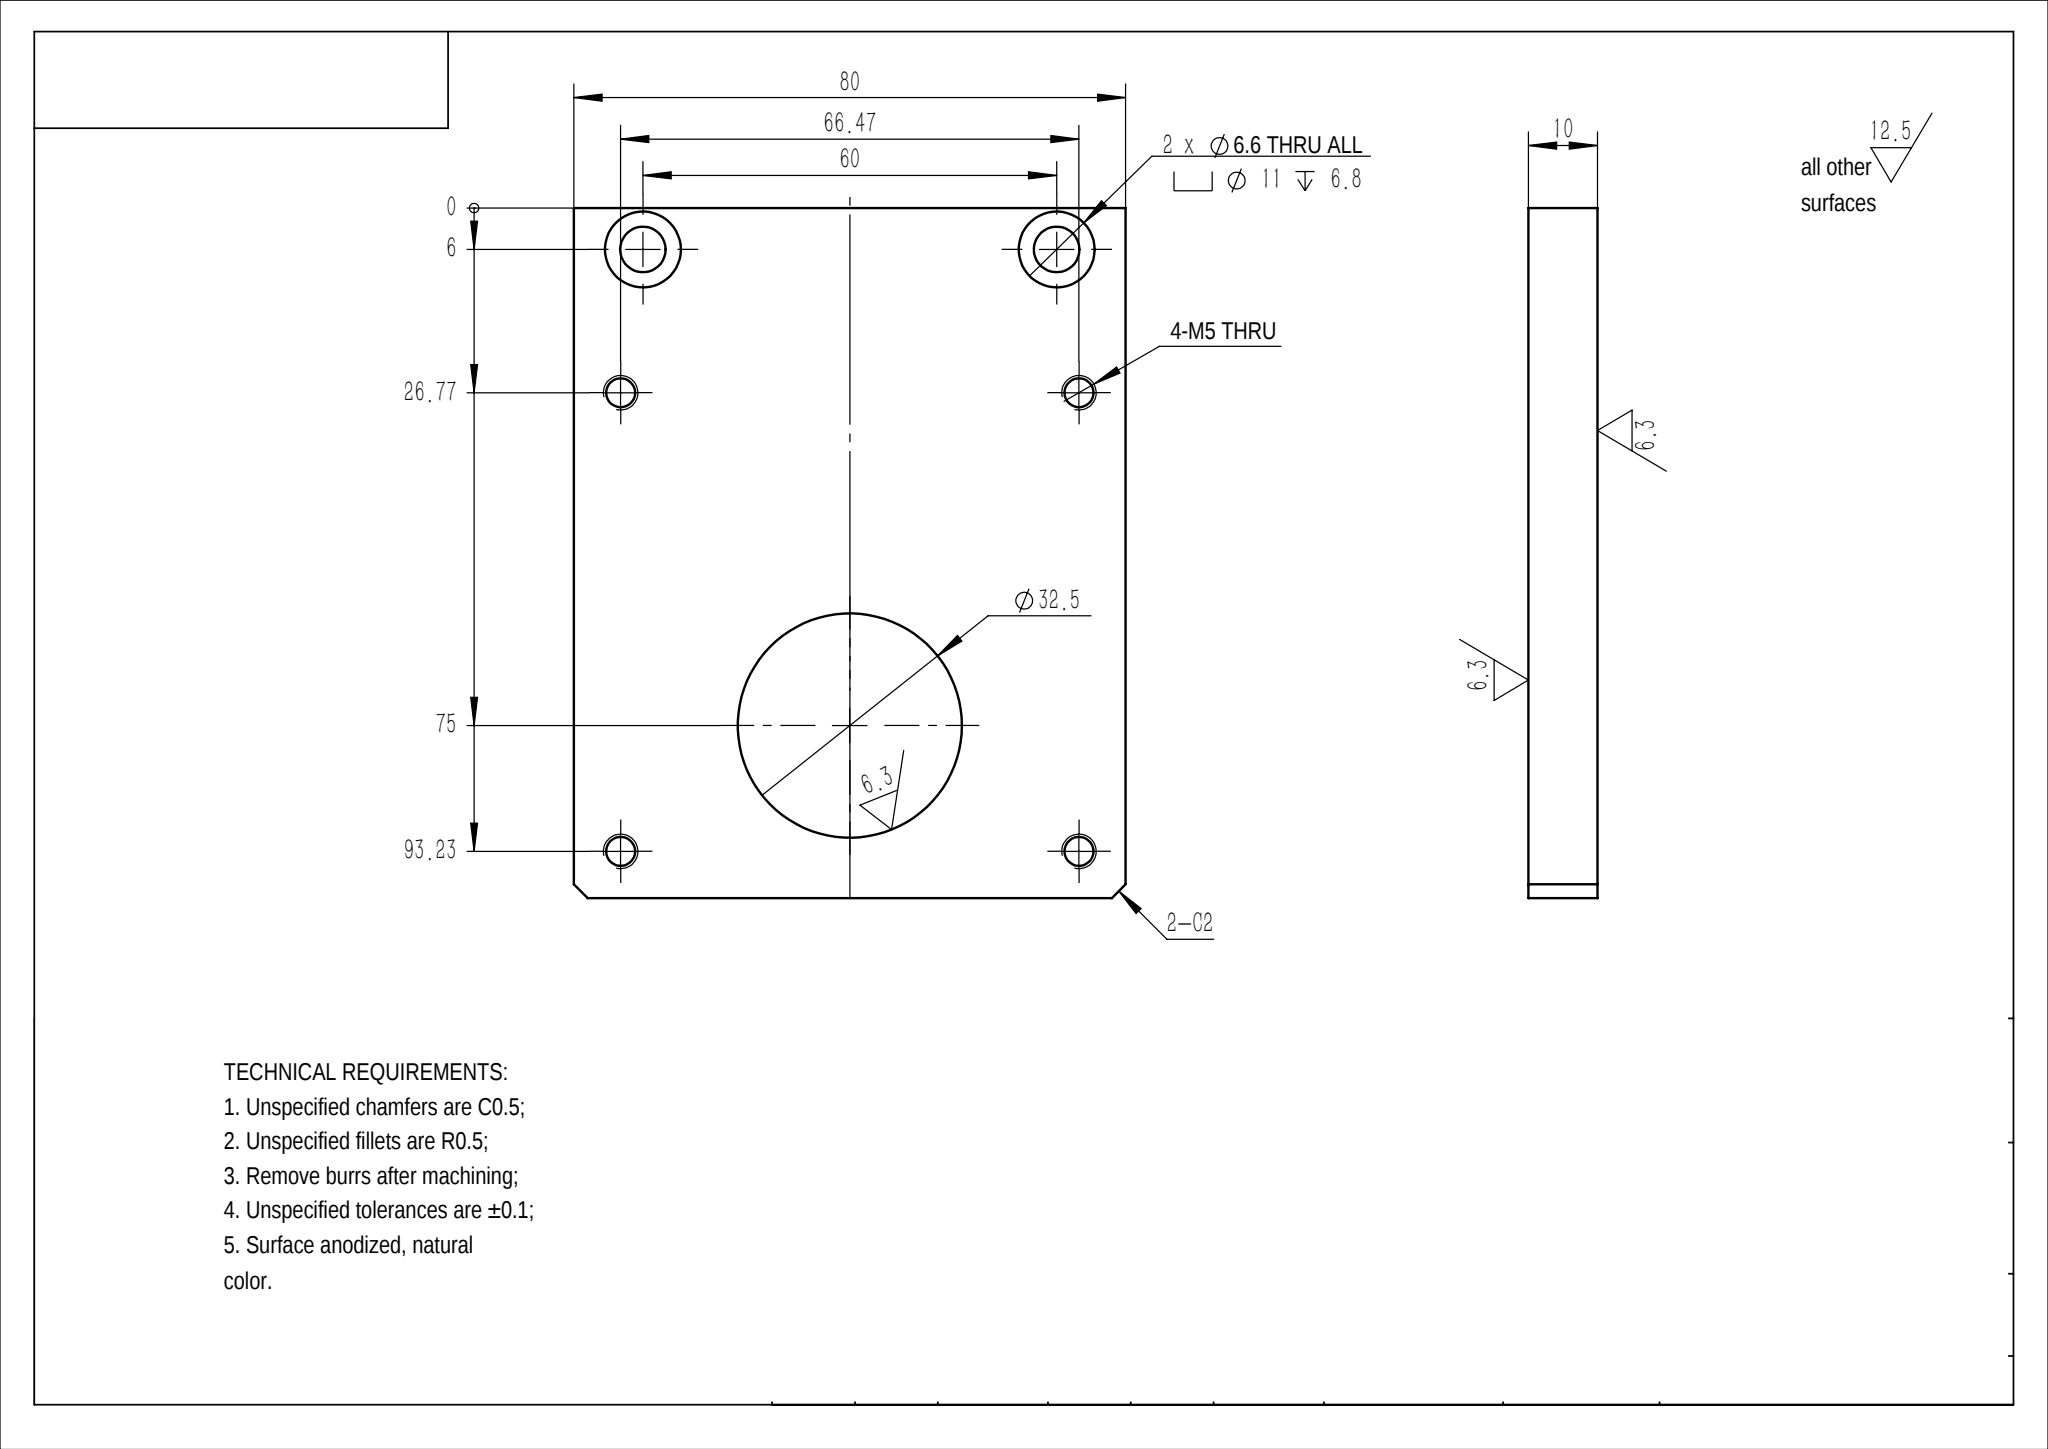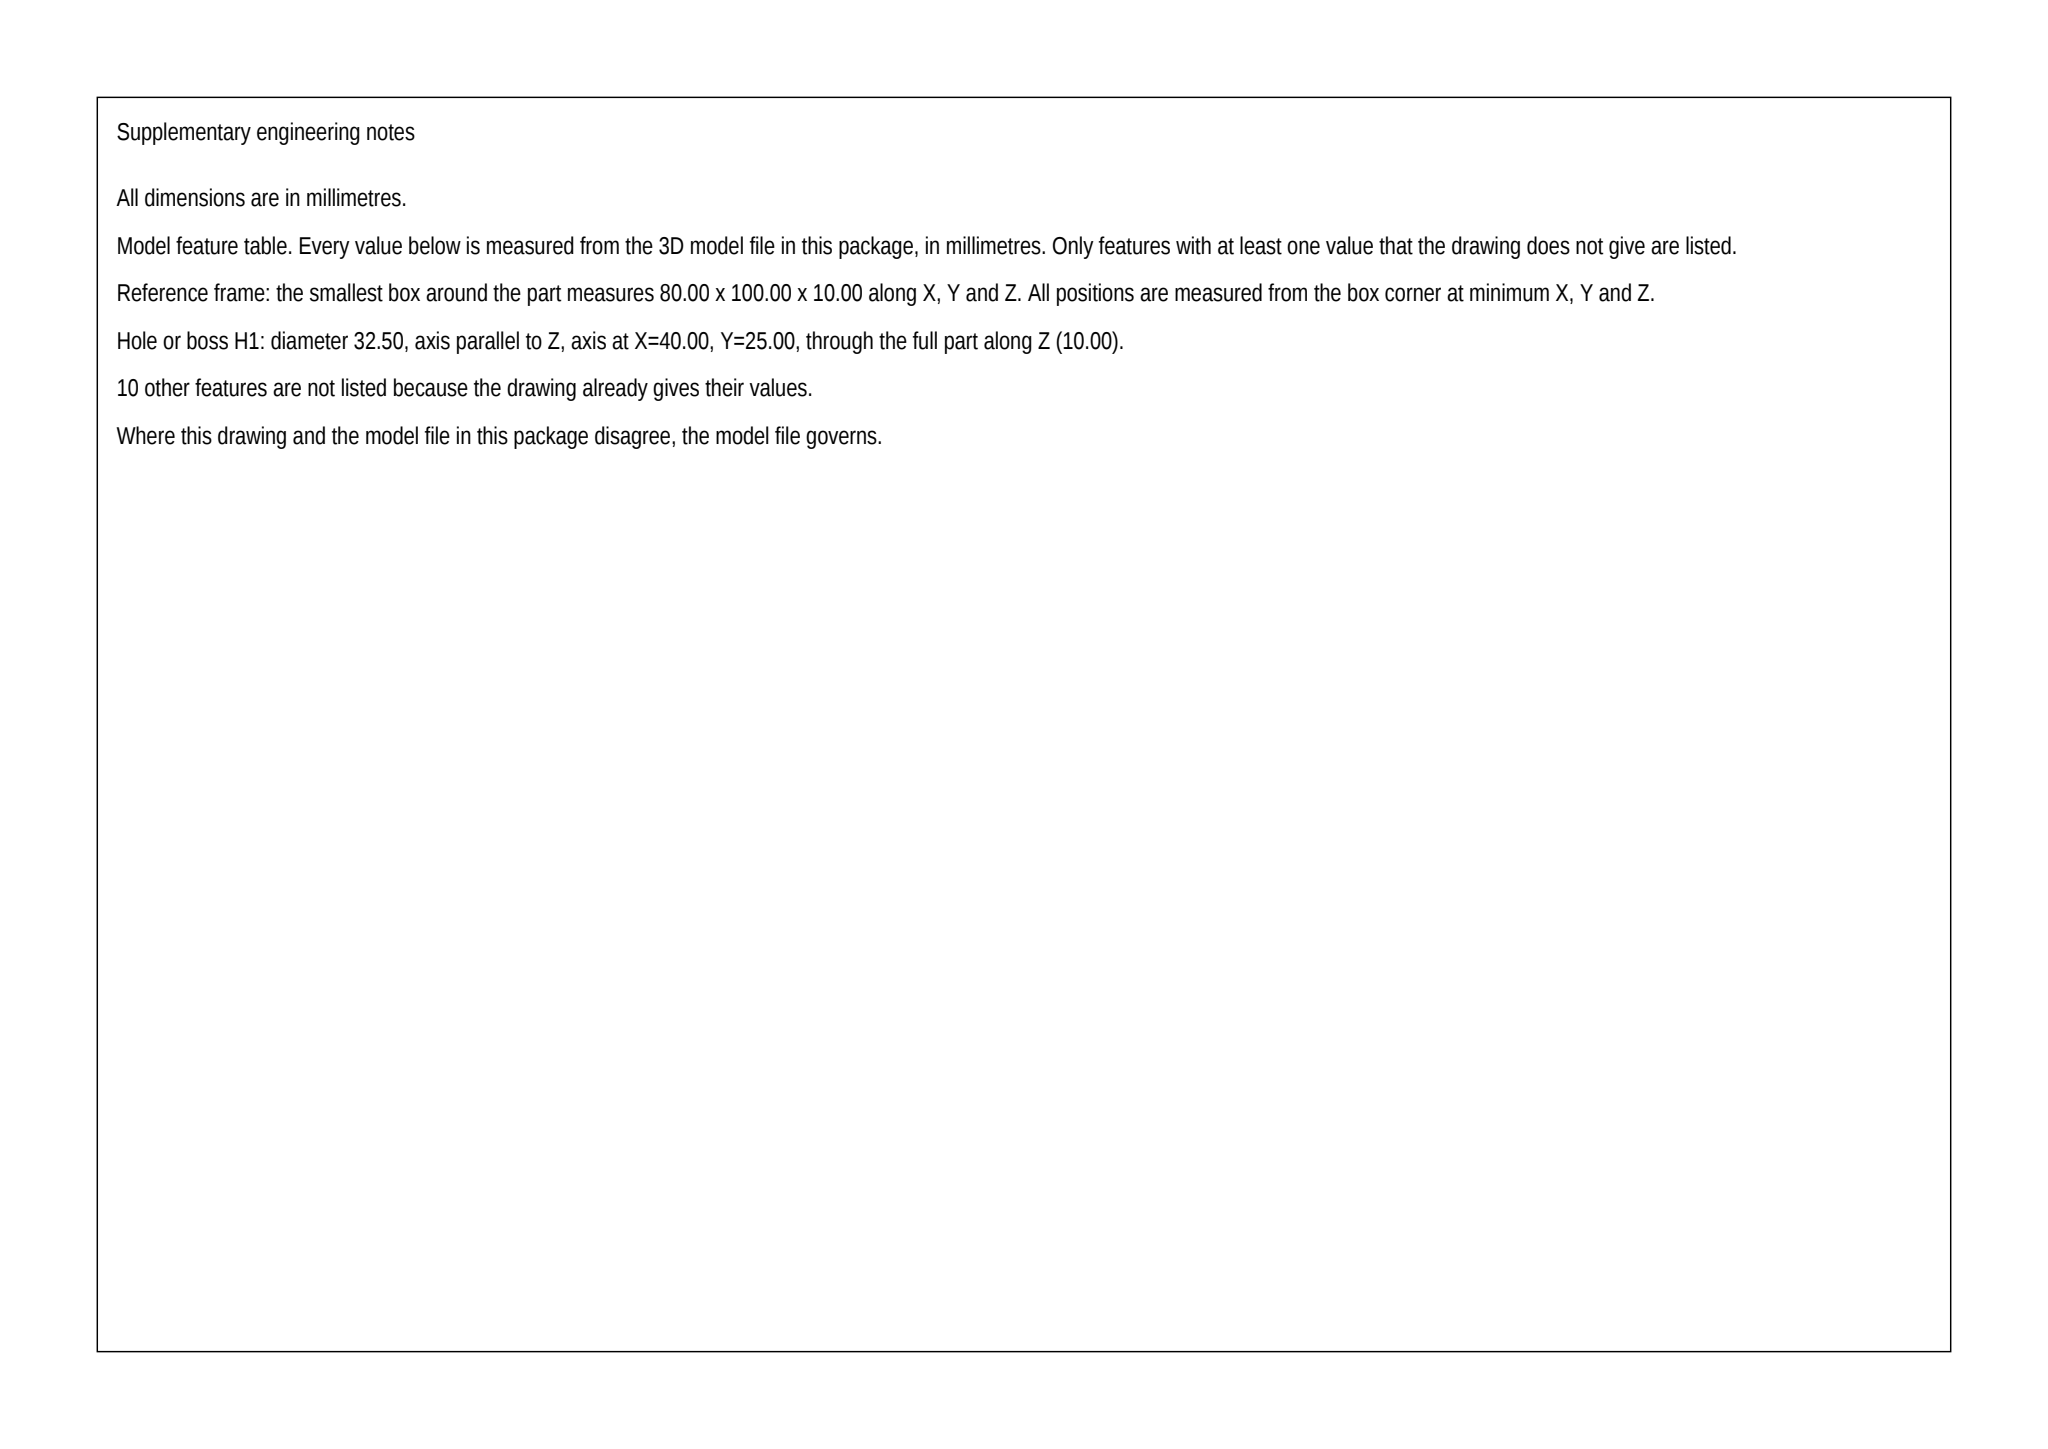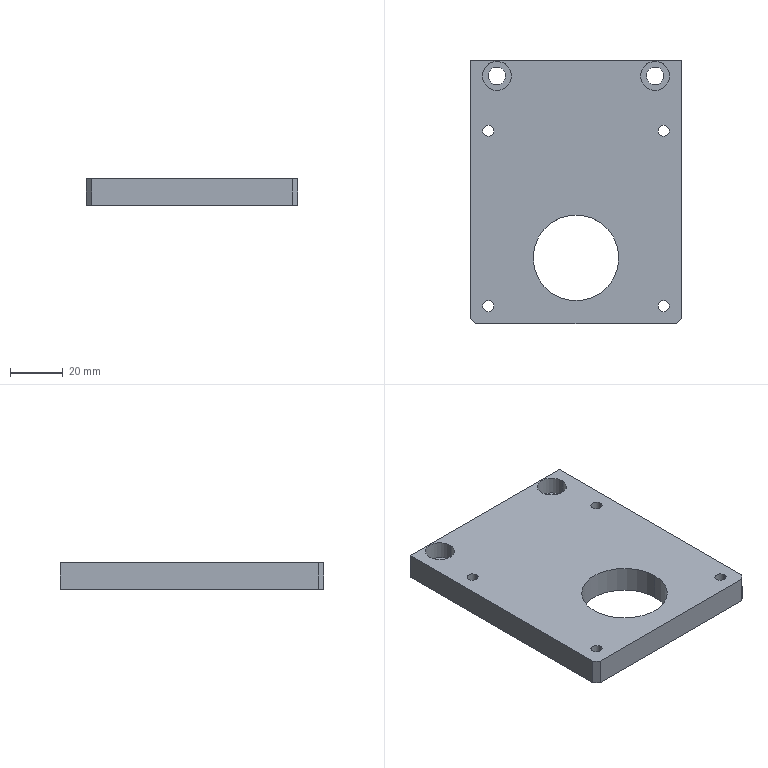Part | SolidWorks | mm | 1 solid | 28 faces | box 80 x 100 x 10 mm | volume 69599 mm3 | cylinder 18 | plane 10 | commonest cylinder face diameters 4.2 x8 11 x4 6.6 x4 32.5 x2
build123d program:
from build123d import *

# Parameters (mm, degrees)
SKETCH1_W                                            = 80
SKETCH1_H                                            = 100
BOSS_EXTRUDE1_DEPTH                                  = 10
SKETCH2_R                                            = 16.25
CUT_EXTRUDE1_DEPTH                                   = 65.807
M5_TAPPED_HOLE1_D                                    = 4.2
CHAMFER1_SIZE                                        = 2
HOLE_SIZE_ACCORDING_TO_TYPE_1_OF_HEXAGON_D           = 6.6
HOLE_SIZE_ACCORDING_TO_TYPE_1_OF_HEXAGON_CBORE_D     = 11
HOLE_SIZE_ACCORDING_TO_TYPE_1_OF_HEXAGON_CBORE_DEPTH = 6.8


with BuildPart() as part:
    # Sketch1 → Boss-Extrude1 (new body)
    with BuildSketch(Plane.XY):
        Rectangle(SKETCH1_W, SKETCH1_H)
    extrude(amount=BOSS_EXTRUDE1_DEPTH)

    # Sketch2 → Cut-Extrude1 (cut, through all)
    with BuildSketch(Plane.XY.offset(10)):
        with Locations((0, -25)):
            Circle(SKETCH2_R)
    extrude(amount=-CUT_EXTRUDE1_DEPTH, mode=Mode.SUBTRACT)

    # M5 Tapped Hole1 (through all)
    with Locations(Plane.XY.offset(10)):
        with Locations((-33.234, 23.234), (-33.234, -43.234), (33.234, -43.234), (33.234, 23.234)):
            Hole(M5_TAPPED_HOLE1_D / 2)

    # Chamfer1
    chamfer1_edges = [part.edges().sort_by_distance(p)[0] for p in [
        (40, -50, 5),
        (-40, -50, 5),
    ]]
    chamfer(chamfer1_edges, length=CHAMFER1_SIZE)

    # Hole Size_According to_Type 1 of Hexagon (through all)
    with Locations(Plane.XY.offset(10)):
        with Locations((-30, 44), (30, 44)):
            CounterBoreHole(HOLE_SIZE_ACCORDING_TO_TYPE_1_OF_HEXAGON_D / 2, HOLE_SIZE_ACCORDING_TO_TYPE_1_OF_HEXAGON_CBORE_D / 2, HOLE_SIZE_ACCORDING_TO_TYPE_1_OF_HEXAGON_CBORE_DEPTH)


solid = part.part
STEP:
#1=CARTESIAN_POINT('',(-35.5,44.,3.2));
#2=VERTEX_POINT('',#1);
#3=CARTESIAN_POINT('',(-24.5,44.,3.2));
#4=VERTEX_POINT('',#3);
#5=CARTESIAN_POINT('',(-30.,44.,3.2));
#6=DIRECTION('',(0.,0.,1.));
#7=DIRECTION('',(1.,0.,0.));
#8=AXIS2_PLACEMENT_3D('',#5,#6,#7);
#9=CIRCLE('',#8,5.5);
#10=EDGE_CURVE('',#2,#4,#9,.T.);
#11=ORIENTED_EDGE('',*,*,#10,.F.);
#12=CARTESIAN_POINT('',(-35.5,44.,10.));
#13=VERTEX_POINT('',#12);
#14=CARTESIAN_POINT('',(-35.5,44.,10.));
#15=DIRECTION('',(0.,0.,1.));
#16=VECTOR('',#15,1000.);
#17=LINE('',#14,#16);
#18=EDGE_CURVE('',#2,#13,#17,.T.);
#19=ORIENTED_EDGE('',*,*,#18,.T.);
#20=CARTESIAN_POINT('',(-24.5,44.,10.));
#21=VERTEX_POINT('',#20);
#22=CARTESIAN_POINT('',(-30.,44.,10.));
#23=DIRECTION('',(0.,0.,1.));
#24=DIRECTION('',(1.,0.,0.));
#25=AXIS2_PLACEMENT_3D('',#22,#23,#24);
#26=CIRCLE('',#25,5.5);
#27=EDGE_CURVE('',#13,#21,#26,.T.);
#28=ORIENTED_EDGE('',*,*,#27,.T.);
#29=CARTESIAN_POINT('',(-24.5,44.,10.));
#30=DIRECTION('',(0.,0.,1.));
#31=VECTOR('',#30,1000.);
#32=LINE('',#29,#31);
#33=EDGE_CURVE('',#4,#21,#32,.T.);
#34=ORIENTED_EDGE('',*,*,#33,.F.);
#35=EDGE_LOOP('',(#11,#19,#28,#34));
#36=FACE_OUTER_BOUND('',#35,.T.);
#37=CARTESIAN_POINT('',(-30.,44.,10.));
#38=DIRECTION('',(0.,0.,1.));
#39=DIRECTION('',(1.,0.,0.));
#40=AXIS2_PLACEMENT_3D('',#37,#38,#39);
#41=CYLINDRICAL_SURFACE('',#40,5.5);
#42=ADVANCED_FACE('',(#36),#41,.F.);
#43=CARTESIAN_POINT('',(-33.3,44.,0.));
#44=VERTEX_POINT('',#43);
#45=CARTESIAN_POINT('',(-26.7,44.,0.));
#46=VERTEX_POINT('',#45);
#47=CARTESIAN_POINT('',(-30.,44.,0.));
#48=DIRECTION('',(0.,0.,1.));
#49=DIRECTION('',(1.,0.,0.));
#50=AXIS2_PLACEMENT_3D('',#47,#48,#49);
#51=CIRCLE('',#50,3.3);
#52=EDGE_CURVE('',#44,#46,#51,.T.);
#53=ORIENTED_EDGE('',*,*,#52,.F.);
#54=CARTESIAN_POINT('',(-33.3,44.,3.2));
#55=VERTEX_POINT('',#54);
#56=CARTESIAN_POINT('',(-33.3,44.,10.));
#57=DIRECTION('',(0.,0.,1.));
#58=VECTOR('',#57,1000.);
#59=LINE('',#56,#58);
#60=EDGE_CURVE('',#44,#55,#59,.T.);
#61=ORIENTED_EDGE('',*,*,#60,.T.);
#62=CARTESIAN_POINT('',(-26.7,44.,3.2));
#63=VERTEX_POINT('',#62);
#64=CARTESIAN_POINT('',(-30.,44.,3.2));
#65=DIRECTION('',(0.,0.,1.));
#66=DIRECTION('',(1.,0.,0.));
#67=AXIS2_PLACEMENT_3D('',#64,#65,#66);
#68=CIRCLE('',#67,3.3);
#69=EDGE_CURVE('',#55,#63,#68,.T.);
#70=ORIENTED_EDGE('',*,*,#69,.T.);
#71=CARTESIAN_POINT('',(-26.7,44.,10.));
#72=DIRECTION('',(0.,0.,1.));
#73=VECTOR('',#72,1000.);
#74=LINE('',#71,#73);
#75=EDGE_CURVE('',#46,#63,#74,.T.);
#76=ORIENTED_EDGE('',*,*,#75,.F.);
#77=EDGE_LOOP('',(#53,#61,#70,#76));
#78=FACE_OUTER_BOUND('',#77,.T.);
#79=CARTESIAN_POINT('',(-30.,44.,10.));
#80=DIRECTION('',(0.,0.,1.));
#81=DIRECTION('',(1.,0.,0.));
#82=AXIS2_PLACEMENT_3D('',#79,#80,#81);
#83=CYLINDRICAL_SURFACE('',#82,3.3);
#84=ADVANCED_FACE('',(#78),#83,.F.);
#85=CARTESIAN_POINT('',(24.5,44.,3.2));
#86=VERTEX_POINT('',#85);
#87=CARTESIAN_POINT('',(35.5,44.,3.2));
#88=VERTEX_POINT('',#87);
#89=CARTESIAN_POINT('',(30.,44.,3.2));
#90=DIRECTION('',(0.,0.,1.));
#91=DIRECTION('',(1.,0.,0.));
#92=AXIS2_PLACEMENT_3D('',#89,#90,#91);
#93=CIRCLE('',#92,5.5);
#94=EDGE_CURVE('',#86,#88,#93,.T.);
#95=ORIENTED_EDGE('',*,*,#94,.F.);
#96=CARTESIAN_POINT('',(24.5,44.,10.));
#97=VERTEX_POINT('',#96);
#98=CARTESIAN_POINT('',(24.5,44.,10.));
#99=DIRECTION('',(0.,0.,1.));
#100=VECTOR('',#99,1000.);
#101=LINE('',#98,#100);
#102=EDGE_CURVE('',#86,#97,#101,.T.);
#103=ORIENTED_EDGE('',*,*,#102,.T.);
#104=CARTESIAN_POINT('',(35.5,44.,10.));
#105=VERTEX_POINT('',#104);
#106=CARTESIAN_POINT('',(30.,44.,10.));
#107=DIRECTION('',(0.,0.,1.));
#108=DIRECTION('',(1.,0.,0.));
#109=AXIS2_PLACEMENT_3D('',#106,#107,#108);
#110=CIRCLE('',#109,5.5);
#111=EDGE_CURVE('',#97,#105,#110,.T.);
#112=ORIENTED_EDGE('',*,*,#111,.T.);
#113=CARTESIAN_POINT('',(35.5,44.,10.));
#114=DIRECTION('',(0.,0.,1.));
#115=VECTOR('',#114,1000.);
#116=LINE('',#113,#115);
#117=EDGE_CURVE('',#88,#105,#116,.T.);
#118=ORIENTED_EDGE('',*,*,#117,.F.);
#119=EDGE_LOOP('',(#95,#103,#112,#118));
#120=FACE_OUTER_BOUND('',#119,.T.);
#121=CARTESIAN_POINT('',(30.,44.,10.));
#122=DIRECTION('',(0.,0.,1.));
#123=DIRECTION('',(1.,0.,0.));
#124=AXIS2_PLACEMENT_3D('',#121,#122,#123);
#125=CYLINDRICAL_SURFACE('',#124,5.5);
#126=ADVANCED_FACE('',(#120),#125,.F.);
#127=CARTESIAN_POINT('',(26.7,44.,0.));
#128=VERTEX_POINT('',#127);
#129=CARTESIAN_POINT('',(33.3,44.,0.));
#130=VERTEX_POINT('',#129);
#131=CARTESIAN_POINT('',(30.,44.,0.));
#132=DIRECTION('',(0.,0.,1.));
#133=DIRECTION('',(1.,0.,0.));
#134=AXIS2_PLACEMENT_3D('',#131,#132,#133);
#135=CIRCLE('',#134,3.3);
#136=EDGE_CURVE('',#128,#130,#135,.T.);
#137=ORIENTED_EDGE('',*,*,#136,.F.);
#138=CARTESIAN_POINT('',(26.7,44.,3.2));
#139=VERTEX_POINT('',#138);
#140=CARTESIAN_POINT('',(26.7,44.,10.));
#141=DIRECTION('',(0.,0.,1.));
#142=VECTOR('',#141,1000.);
#143=LINE('',#140,#142);
#144=EDGE_CURVE('',#128,#139,#143,.T.);
#145=ORIENTED_EDGE('',*,*,#144,.T.);
#146=CARTESIAN_POINT('',(33.3,44.,3.2));
#147=VERTEX_POINT('',#146);
#148=CARTESIAN_POINT('',(30.,44.,3.2));
#149=DIRECTION('',(0.,0.,1.));
#150=DIRECTION('',(1.,0.,0.));
#151=AXIS2_PLACEMENT_3D('',#148,#149,#150);
#152=CIRCLE('',#151,3.3);
#153=EDGE_CURVE('',#139,#147,#152,.T.);
#154=ORIENTED_EDGE('',*,*,#153,.T.);
#155=CARTESIAN_POINT('',(33.3,44.,10.));
#156=DIRECTION('',(0.,0.,1.));
#157=VECTOR('',#156,1000.);
#158=LINE('',#155,#157);
#159=EDGE_CURVE('',#130,#147,#158,.T.);
#160=ORIENTED_EDGE('',*,*,#159,.F.);
#161=EDGE_LOOP('',(#137,#145,#154,#160));
#162=FACE_OUTER_BOUND('',#161,.T.);
#163=CARTESIAN_POINT('',(30.,44.,10.));
#164=DIRECTION('',(0.,0.,1.));
#165=DIRECTION('',(1.,0.,0.));
#166=AXIS2_PLACEMENT_3D('',#163,#164,#165);
#167=CYLINDRICAL_SURFACE('',#166,3.3);
#168=ADVANCED_FACE('',(#162),#167,.F.);
#169=CARTESIAN_POINT('',(-35.334,23.234,0.));
#170=VERTEX_POINT('',#169);
#171=CARTESIAN_POINT('',(-31.134,23.234,0.));
#172=VERTEX_POINT('',#171);
#173=CARTESIAN_POINT('',(-33.234,23.234,0.));
#174=DIRECTION('',(0.,0.,1.));
#175=DIRECTION('',(1.,0.,0.));
#176=AXIS2_PLACEMENT_3D('',#173,#174,#175);
#177=CIRCLE('',#176,2.1);
#178=EDGE_CURVE('',#170,#172,#177,.T.);
#179=ORIENTED_EDGE('',*,*,#178,.F.);
#180=CARTESIAN_POINT('',(-35.334,23.234,10.));
#181=VERTEX_POINT('',#180);
#182=CARTESIAN_POINT('',(-35.334,23.234,10.));
#183=DIRECTION('',(0.,0.,1.));
#184=VECTOR('',#183,1000.);
#185=LINE('',#182,#184);
#186=EDGE_CURVE('',#170,#181,#185,.T.);
#187=ORIENTED_EDGE('',*,*,#186,.T.);
#188=CARTESIAN_POINT('',(-31.134,23.234,10.));
#189=VERTEX_POINT('',#188);
#190=CARTESIAN_POINT('',(-33.234,23.234,10.));
#191=DIRECTION('',(0.,0.,1.));
#192=DIRECTION('',(1.,0.,0.));
#193=AXIS2_PLACEMENT_3D('',#190,#191,#192);
#194=CIRCLE('',#193,2.1);
#195=EDGE_CURVE('',#181,#189,#194,.T.);
#196=ORIENTED_EDGE('',*,*,#195,.T.);
#197=CARTESIAN_POINT('',(-31.134,23.234,10.));
#198=DIRECTION('',(0.,0.,1.));
#199=VECTOR('',#198,1000.);
#200=LINE('',#197,#199);
#201=EDGE_CURVE('',#172,#189,#200,.T.);
#202=ORIENTED_EDGE('',*,*,#201,.F.);
#203=EDGE_LOOP('',(#179,#187,#196,#202));
#204=FACE_OUTER_BOUND('',#203,.T.);
#205=CARTESIAN_POINT('',(-33.234,23.234,10.));
#206=DIRECTION('',(0.,0.,1.));
#207=DIRECTION('',(1.,0.,0.));
#208=AXIS2_PLACEMENT_3D('',#205,#206,#207);
#209=CYLINDRICAL_SURFACE('',#208,2.1);
#210=ADVANCED_FACE('',(#204),#209,.F.);
#211=CARTESIAN_POINT('',(-35.334,-43.234,0.));
#212=VERTEX_POINT('',#211);
#213=CARTESIAN_POINT('',(-31.134,-43.234,0.));
#214=VERTEX_POINT('',#213);
#215=CARTESIAN_POINT('',(-33.234,-43.234,0.));
#216=DIRECTION('',(0.,0.,1.));
#217=DIRECTION('',(1.,0.,0.));
#218=AXIS2_PLACEMENT_3D('',#215,#216,#217);
#219=CIRCLE('',#218,2.1);
#220=EDGE_CURVE('',#212,#214,#219,.T.);
#221=ORIENTED_EDGE('',*,*,#220,.F.);
#222=CARTESIAN_POINT('',(-35.334,-43.234,10.));
#223=VERTEX_POINT('',#222);
#224=CARTESIAN_POINT('',(-35.334,-43.234,10.));
#225=DIRECTION('',(0.,0.,1.));
#226=VECTOR('',#225,1000.);
#227=LINE('',#224,#226);
#228=EDGE_CURVE('',#212,#223,#227,.T.);
#229=ORIENTED_EDGE('',*,*,#228,.T.);
#230=CARTESIAN_POINT('',(-31.134,-43.234,10.));
#231=VERTEX_POINT('',#230);
#232=CARTESIAN_POINT('',(-33.234,-43.234,10.));
#233=DIRECTION('',(0.,0.,1.));
#234=DIRECTION('',(1.,0.,0.));
#235=AXIS2_PLACEMENT_3D('',#232,#233,#234);
#236=CIRCLE('',#235,2.1);
#237=EDGE_CURVE('',#223,#231,#236,.T.);
#238=ORIENTED_EDGE('',*,*,#237,.T.);
#239=CARTESIAN_POINT('',(-31.134,-43.234,10.));
#240=DIRECTION('',(0.,0.,1.));
#241=VECTOR('',#240,1000.);
#242=LINE('',#239,#241);
#243=EDGE_CURVE('',#214,#231,#242,.T.);
#244=ORIENTED_EDGE('',*,*,#243,.F.);
#245=EDGE_LOOP('',(#221,#229,#238,#244));
#246=FACE_OUTER_BOUND('',#245,.T.);
#247=CARTESIAN_POINT('',(-33.234,-43.234,10.));
#248=DIRECTION('',(0.,0.,1.));
#249=DIRECTION('',(1.,0.,0.));
#250=AXIS2_PLACEMENT_3D('',#247,#248,#249);
#251=CYLINDRICAL_SURFACE('',#250,2.1);
#252=ADVANCED_FACE('',(#246),#251,.F.);
#253=CARTESIAN_POINT('',(31.134,-43.234,0.));
#254=VERTEX_POINT('',#253);
#255=CARTESIAN_POINT('',(35.334,-43.234,0.));
#256=VERTEX_POINT('',#255);
#257=CARTESIAN_POINT('',(33.234,-43.234,0.));
#258=DIRECTION('',(0.,0.,1.));
#259=DIRECTION('',(1.,0.,0.));
#260=AXIS2_PLACEMENT_3D('',#257,#258,#259);
#261=CIRCLE('',#260,2.1);
#262=EDGE_CURVE('',#254,#256,#261,.T.);
#263=ORIENTED_EDGE('',*,*,#262,.F.);
#264=CARTESIAN_POINT('',(31.134,-43.234,10.));
#265=VERTEX_POINT('',#264);
#266=CARTESIAN_POINT('',(31.134,-43.234,10.));
#267=DIRECTION('',(0.,0.,1.));
#268=VECTOR('',#267,1000.);
#269=LINE('',#266,#268);
#270=EDGE_CURVE('',#254,#265,#269,.T.);
#271=ORIENTED_EDGE('',*,*,#270,.T.);
#272=CARTESIAN_POINT('',(35.334,-43.234,10.));
#273=VERTEX_POINT('',#272);
#274=CARTESIAN_POINT('',(33.234,-43.234,10.));
#275=DIRECTION('',(0.,0.,1.));
#276=DIRECTION('',(1.,0.,0.));
#277=AXIS2_PLACEMENT_3D('',#274,#275,#276);
#278=CIRCLE('',#277,2.1);
#279=EDGE_CURVE('',#265,#273,#278,.T.);
#280=ORIENTED_EDGE('',*,*,#279,.T.);
#281=CARTESIAN_POINT('',(35.334,-43.234,10.));
#282=DIRECTION('',(0.,0.,1.));
#283=VECTOR('',#282,1000.);
#284=LINE('',#281,#283);
#285=EDGE_CURVE('',#256,#273,#284,.T.);
#286=ORIENTED_EDGE('',*,*,#285,.F.);
#287=EDGE_LOOP('',(#263,#271,#280,#286));
#288=FACE_OUTER_BOUND('',#287,.T.);
#289=CARTESIAN_POINT('',(33.234,-43.234,10.));
#290=DIRECTION('',(0.,0.,1.));
#291=DIRECTION('',(1.,0.,0.));
#292=AXIS2_PLACEMENT_3D('',#289,#290,#291);
#293=CYLINDRICAL_SURFACE('',#292,2.1);
#294=ADVANCED_FACE('',(#288),#293,.F.);
#295=CARTESIAN_POINT('',(31.134,23.234,0.));
#296=VERTEX_POINT('',#295);
#297=CARTESIAN_POINT('',(35.334,23.234,0.));
#298=VERTEX_POINT('',#297);
#299=CARTESIAN_POINT('',(33.234,23.234,0.));
#300=DIRECTION('',(0.,0.,1.));
#301=DIRECTION('',(1.,0.,0.));
#302=AXIS2_PLACEMENT_3D('',#299,#300,#301);
#303=CIRCLE('',#302,2.1);
#304=EDGE_CURVE('',#296,#298,#303,.T.);
#305=ORIENTED_EDGE('',*,*,#304,.F.);
#306=CARTESIAN_POINT('',(31.134,23.234,10.));
#307=VERTEX_POINT('',#306);
#308=CARTESIAN_POINT('',(31.134,23.234,10.));
#309=DIRECTION('',(0.,0.,1.));
#310=VECTOR('',#309,1000.);
#311=LINE('',#308,#310);
#312=EDGE_CURVE('',#296,#307,#311,.T.);
#313=ORIENTED_EDGE('',*,*,#312,.T.);
#314=CARTESIAN_POINT('',(35.334,23.234,10.));
#315=VERTEX_POINT('',#314);
#316=CARTESIAN_POINT('',(33.234,23.234,10.));
#317=DIRECTION('',(0.,0.,1.));
#318=DIRECTION('',(1.,0.,0.));
#319=AXIS2_PLACEMENT_3D('',#316,#317,#318);
#320=CIRCLE('',#319,2.1);
#321=EDGE_CURVE('',#307,#315,#320,.T.);
#322=ORIENTED_EDGE('',*,*,#321,.T.);
#323=CARTESIAN_POINT('',(35.334,23.234,10.));
#324=DIRECTION('',(0.,0.,1.));
#325=VECTOR('',#324,1000.);
#326=LINE('',#323,#325);
#327=EDGE_CURVE('',#298,#315,#326,.T.);
#328=ORIENTED_EDGE('',*,*,#327,.F.);
#329=EDGE_LOOP('',(#305,#313,#322,#328));
#330=FACE_OUTER_BOUND('',#329,.T.);
#331=CARTESIAN_POINT('',(33.234,23.234,10.));
#332=DIRECTION('',(0.,0.,1.));
#333=DIRECTION('',(1.,0.,0.));
#334=AXIS2_PLACEMENT_3D('',#331,#332,#333);
#335=CYLINDRICAL_SURFACE('',#334,2.1);
#336=ADVANCED_FACE('',(#330),#335,.F.);
#337=CARTESIAN_POINT('',(-16.25,-25.,0.));
#338=VERTEX_POINT('',#337);
#339=CARTESIAN_POINT('',(16.25,-25.,0.));
#340=VERTEX_POINT('',#339);
#341=CARTESIAN_POINT('',(0.,-25.,0.));
#342=DIRECTION('',(0.,0.,1.));
#343=DIRECTION('',(1.,0.,0.));
#344=AXIS2_PLACEMENT_3D('',#341,#342,#343);
#345=CIRCLE('',#344,16.25);
#346=EDGE_CURVE('',#338,#340,#345,.T.);
#347=ORIENTED_EDGE('',*,*,#346,.F.);
#348=CARTESIAN_POINT('',(-16.25,-25.,10.));
#349=VERTEX_POINT('',#348);
#350=CARTESIAN_POINT('',(-16.25,-25.,0.));
#351=DIRECTION('',(0.,0.,1.));
#352=VECTOR('',#351,1000.);
#353=LINE('',#350,#352);
#354=EDGE_CURVE('',#338,#349,#353,.T.);
#355=ORIENTED_EDGE('',*,*,#354,.T.);
#356=CARTESIAN_POINT('',(16.25,-25.,10.));
#357=VERTEX_POINT('',#356);
#358=CARTESIAN_POINT('',(0.,-25.,10.));
#359=DIRECTION('',(0.,0.,1.));
#360=DIRECTION('',(1.,0.,0.));
#361=AXIS2_PLACEMENT_3D('',#358,#359,#360);
#362=CIRCLE('',#361,16.25);
#363=EDGE_CURVE('',#349,#357,#362,.T.);
#364=ORIENTED_EDGE('',*,*,#363,.T.);
#365=CARTESIAN_POINT('',(16.25,-25.,0.));
#366=DIRECTION('',(0.,0.,1.));
#367=VECTOR('',#366,1000.);
#368=LINE('',#365,#367);
#369=EDGE_CURVE('',#340,#357,#368,.T.);
#370=ORIENTED_EDGE('',*,*,#369,.F.);
#371=EDGE_LOOP('',(#347,#355,#364,#370));
#372=FACE_OUTER_BOUND('',#371,.T.);
#373=CARTESIAN_POINT('',(0.,-25.,0.));
#374=DIRECTION('',(0.,0.,1.));
#375=DIRECTION('',(1.,0.,0.));
#376=AXIS2_PLACEMENT_3D('',#373,#374,#375);
#377=CYLINDRICAL_SURFACE('',#376,16.25);
#378=ADVANCED_FACE('',(#372),#377,.F.);
#379=CARTESIAN_POINT('',(-40.,50.,0.));
#380=VERTEX_POINT('',#379);
#381=CARTESIAN_POINT('',(-40.,-48.,0.));
#382=VERTEX_POINT('',#381);
#383=CARTESIAN_POINT('',(-40.,-50.,0.));
#384=DIRECTION('',(0.,-1.,0.));
#385=VECTOR('',#384,1000.);
#386=LINE('',#383,#385);
#387=EDGE_CURVE('',#380,#382,#386,.T.);
#388=ORIENTED_EDGE('',*,*,#387,.T.);
#389=CARTESIAN_POINT('',(-40.,-48.,10.));
#390=VERTEX_POINT('',#389);
#391=CARTESIAN_POINT('',(-40.,-48.,10.));
#392=DIRECTION('',(0.,0.,1.));
#393=VECTOR('',#392,1000.);
#394=LINE('',#391,#393);
#395=EDGE_CURVE('',#382,#390,#394,.T.);
#396=ORIENTED_EDGE('',*,*,#395,.T.);
#397=CARTESIAN_POINT('',(-40.,50.,10.));
#398=VERTEX_POINT('',#397);
#399=CARTESIAN_POINT('',(-40.,-50.,10.));
#400=DIRECTION('',(0.,-1.,0.));
#401=VECTOR('',#400,1000.);
#402=LINE('',#399,#401);
#403=EDGE_CURVE('',#398,#390,#402,.T.);
#404=ORIENTED_EDGE('',*,*,#403,.F.);
#405=CARTESIAN_POINT('',(-40.,50.,10.));
#406=DIRECTION('',(0.,0.,-1.));
#407=VECTOR('',#406,1000.);
#408=LINE('',#405,#407);
#409=EDGE_CURVE('',#398,#380,#408,.T.);
#410=ORIENTED_EDGE('',*,*,#409,.T.);
#411=EDGE_LOOP('',(#388,#396,#404,#410));
#412=FACE_OUTER_BOUND('',#411,.T.);
#413=CARTESIAN_POINT('',(-40.,-50.,10.));
#414=DIRECTION('',(1.,0.,0.));
#415=DIRECTION('',(0.,0.,-1.));
#416=AXIS2_PLACEMENT_3D('',#413,#414,#415);
#417=PLANE('',#416);
#418=ADVANCED_FACE('',(#412),#417,.F.);
#419=CARTESIAN_POINT('',(-38.,-50.,0.));
#420=VERTEX_POINT('',#419);
#421=CARTESIAN_POINT('',(38.,-50.,0.));
#422=VERTEX_POINT('',#421);
#423=CARTESIAN_POINT('',(40.,-50.,0.));
#424=DIRECTION('',(1.,0.,0.));
#425=VECTOR('',#424,1000.);
#426=LINE('',#423,#425);
#427=EDGE_CURVE('',#420,#422,#426,.T.);
#428=ORIENTED_EDGE('',*,*,#427,.T.);
#429=CARTESIAN_POINT('',(38.,-50.,10.));
#430=VERTEX_POINT('',#429);
#431=CARTESIAN_POINT('',(38.,-50.,10.));
#432=DIRECTION('',(0.,0.,1.));
#433=VECTOR('',#432,1000.);
#434=LINE('',#431,#433);
#435=EDGE_CURVE('',#422,#430,#434,.T.);
#436=ORIENTED_EDGE('',*,*,#435,.T.);
#437=CARTESIAN_POINT('',(-38.,-50.,10.));
#438=VERTEX_POINT('',#437);
#439=CARTESIAN_POINT('',(40.,-50.,10.));
#440=DIRECTION('',(1.,0.,0.));
#441=VECTOR('',#440,1000.);
#442=LINE('',#439,#441);
#443=EDGE_CURVE('',#438,#430,#442,.T.);
#444=ORIENTED_EDGE('',*,*,#443,.F.);
#445=CARTESIAN_POINT('',(-38.,-50.,10.));
#446=DIRECTION('',(0.,0.,-1.));
#447=VECTOR('',#446,1000.);
#448=LINE('',#445,#447);
#449=EDGE_CURVE('',#438,#420,#448,.T.);
#450=ORIENTED_EDGE('',*,*,#449,.T.);
#451=EDGE_LOOP('',(#428,#436,#444,#450));
#452=FACE_OUTER_BOUND('',#451,.T.);
#453=CARTESIAN_POINT('',(40.,-50.,10.));
#454=DIRECTION('',(-0.,1.,0.));
#455=DIRECTION('',(-1.,-0.,0.));
#456=AXIS2_PLACEMENT_3D('',#453,#454,#455);
#457=PLANE('',#456);
#458=ADVANCED_FACE('',(#452),#457,.F.);
#459=CARTESIAN_POINT('',(40.,-48.,10.));
#460=VERTEX_POINT('',#459);
#461=CARTESIAN_POINT('',(40.,50.,10.));
#462=VERTEX_POINT('',#461);
#463=CARTESIAN_POINT('',(40.,-50.,10.));
#464=DIRECTION('',(0.,1.,0.));
#465=VECTOR('',#464,1000.);
#466=LINE('',#463,#465);
#467=EDGE_CURVE('',#460,#462,#466,.T.);
#468=ORIENTED_EDGE('',*,*,#467,.F.);
#469=CARTESIAN_POINT('',(40.,-48.,0.));
#470=VERTEX_POINT('',#469);
#471=CARTESIAN_POINT('',(40.,-48.,10.));
#472=DIRECTION('',(0.,0.,-1.));
#473=VECTOR('',#472,1000.);
#474=LINE('',#471,#473);
#475=EDGE_CURVE('',#460,#470,#474,.T.);
#476=ORIENTED_EDGE('',*,*,#475,.T.);
#477=CARTESIAN_POINT('',(40.,50.,0.));
#478=VERTEX_POINT('',#477);
#479=CARTESIAN_POINT('',(40.,-50.,0.));
#480=DIRECTION('',(0.,1.,0.));
#481=VECTOR('',#480,1000.);
#482=LINE('',#479,#481);
#483=EDGE_CURVE('',#470,#478,#482,.T.);
#484=ORIENTED_EDGE('',*,*,#483,.T.);
#485=CARTESIAN_POINT('',(40.,50.,10.));
#486=DIRECTION('',(0.,0.,-1.));
#487=VECTOR('',#486,1000.);
#488=LINE('',#485,#487);
#489=EDGE_CURVE('',#462,#478,#488,.T.);
#490=ORIENTED_EDGE('',*,*,#489,.F.);
#491=EDGE_LOOP('',(#468,#476,#484,#490));
#492=FACE_OUTER_BOUND('',#491,.T.);
#493=CARTESIAN_POINT('',(40.,-50.,10.));
#494=DIRECTION('',(-1.,0.,0.));
#495=DIRECTION('',(0.,0.,1.));
#496=AXIS2_PLACEMENT_3D('',#493,#494,#495);
#497=PLANE('',#496);
#498=ADVANCED_FACE('',(#492),#497,.F.);
#499=CARTESIAN_POINT('',(40.,50.,0.));
#500=DIRECTION('',(-1.,-0.,0.));
#501=VECTOR('',#500,1000.);
#502=LINE('',#499,#501);
#503=EDGE_CURVE('',#478,#380,#502,.T.);
#504=ORIENTED_EDGE('',*,*,#503,.T.);
#505=ORIENTED_EDGE('',*,*,#409,.F.);
#506=CARTESIAN_POINT('',(40.,50.,10.));
#507=DIRECTION('',(-1.,-0.,0.));
#508=VECTOR('',#507,1000.);
#509=LINE('',#506,#508);
#510=EDGE_CURVE('',#462,#398,#509,.T.);
#511=ORIENTED_EDGE('',*,*,#510,.F.);
#512=ORIENTED_EDGE('',*,*,#489,.T.);
#513=EDGE_LOOP('',(#504,#505,#511,#512));
#514=FACE_OUTER_BOUND('',#513,.T.);
#515=CARTESIAN_POINT('',(40.,50.,10.));
#516=DIRECTION('',(0.,-1.,0.));
#517=DIRECTION('',(1.,0.,0.));
#518=AXIS2_PLACEMENT_3D('',#515,#516,#517);
#519=PLANE('',#518);
#520=ADVANCED_FACE('',(#514),#519,.F.);
#521=CARTESIAN_POINT('',(-30.,44.,10.));
#522=DIRECTION('',(0.,0.,1.));
#523=DIRECTION('',(1.,0.,0.));
#524=AXIS2_PLACEMENT_3D('',#521,#522,#523);
#525=CIRCLE('',#524,5.5);
#526=EDGE_CURVE('',#21,#13,#525,.T.);
#527=ORIENTED_EDGE('',*,*,#526,.F.);
#528=ORIENTED_EDGE('',*,*,#27,.F.);
#529=EDGE_LOOP('',(#527,#528));
#530=FACE_BOUND('',#529,.T.);
#531=CARTESIAN_POINT('',(30.,44.,10.));
#532=DIRECTION('',(0.,0.,1.));
#533=DIRECTION('',(1.,0.,0.));
#534=AXIS2_PLACEMENT_3D('',#531,#532,#533);
#535=CIRCLE('',#534,5.5);
#536=EDGE_CURVE('',#105,#97,#535,.T.);
#537=ORIENTED_EDGE('',*,*,#536,.F.);
#538=ORIENTED_EDGE('',*,*,#111,.F.);
#539=EDGE_LOOP('',(#537,#538));
#540=FACE_BOUND('',#539,.T.);
#541=CARTESIAN_POINT('',(-33.234,23.234,10.));
#542=DIRECTION('',(0.,0.,1.));
#543=DIRECTION('',(1.,0.,0.));
#544=AXIS2_PLACEMENT_3D('',#541,#542,#543);
#545=CIRCLE('',#544,2.1);
#546=EDGE_CURVE('',#189,#181,#545,.T.);
#547=ORIENTED_EDGE('',*,*,#546,.F.);
#548=ORIENTED_EDGE('',*,*,#195,.F.);
#549=EDGE_LOOP('',(#547,#548));
#550=FACE_BOUND('',#549,.T.);
#551=CARTESIAN_POINT('',(-33.234,-43.234,10.));
#552=DIRECTION('',(0.,0.,1.));
#553=DIRECTION('',(1.,0.,0.));
#554=AXIS2_PLACEMENT_3D('',#551,#552,#553);
#555=CIRCLE('',#554,2.1);
#556=EDGE_CURVE('',#231,#223,#555,.T.);
#557=ORIENTED_EDGE('',*,*,#556,.F.);
#558=ORIENTED_EDGE('',*,*,#237,.F.);
#559=EDGE_LOOP('',(#557,#558));
#560=FACE_BOUND('',#559,.T.);
#561=CARTESIAN_POINT('',(33.234,-43.234,10.));
#562=DIRECTION('',(0.,0.,1.));
#563=DIRECTION('',(1.,0.,0.));
#564=AXIS2_PLACEMENT_3D('',#561,#562,#563);
#565=CIRCLE('',#564,2.1);
#566=EDGE_CURVE('',#273,#265,#565,.T.);
#567=ORIENTED_EDGE('',*,*,#566,.F.);
#568=ORIENTED_EDGE('',*,*,#279,.F.);
#569=EDGE_LOOP('',(#567,#568));
#570=FACE_BOUND('',#569,.T.);
#571=CARTESIAN_POINT('',(33.234,23.234,10.));
#572=DIRECTION('',(0.,0.,1.));
#573=DIRECTION('',(1.,0.,0.));
#574=AXIS2_PLACEMENT_3D('',#571,#572,#573);
#575=CIRCLE('',#574,2.1);
#576=EDGE_CURVE('',#315,#307,#575,.T.);
#577=ORIENTED_EDGE('',*,*,#576,.F.);
#578=ORIENTED_EDGE('',*,*,#321,.F.);
#579=EDGE_LOOP('',(#577,#578));
#580=FACE_BOUND('',#579,.T.);
#581=CARTESIAN_POINT('',(0.,-25.,10.));
#582=DIRECTION('',(0.,0.,1.));
#583=DIRECTION('',(1.,0.,0.));
#584=AXIS2_PLACEMENT_3D('',#581,#582,#583);
#585=CIRCLE('',#584,16.25);
#586=EDGE_CURVE('',#357,#349,#585,.T.);
#587=ORIENTED_EDGE('',*,*,#586,.F.);
#588=ORIENTED_EDGE('',*,*,#363,.F.);
#589=EDGE_LOOP('',(#587,#588));
#590=FACE_BOUND('',#589,.T.);
#591=ORIENTED_EDGE('',*,*,#443,.T.);
#592=CARTESIAN_POINT('',(44.,-44.,10.));
#593=DIRECTION('',(0.7071,0.7071,0.));
#594=VECTOR('',#593,1000.);
#595=LINE('',#592,#594);
#596=EDGE_CURVE('',#430,#460,#595,.T.);
#597=ORIENTED_EDGE('',*,*,#596,.T.);
#598=ORIENTED_EDGE('',*,*,#467,.T.);
#599=ORIENTED_EDGE('',*,*,#510,.T.);
#600=ORIENTED_EDGE('',*,*,#403,.T.);
#601=CARTESIAN_POINT('',(-44.,-44.,10.));
#602=DIRECTION('',(0.7071,-0.7071,0.));
#603=VECTOR('',#602,1000.);
#604=LINE('',#601,#603);
#605=EDGE_CURVE('',#390,#438,#604,.T.);
#606=ORIENTED_EDGE('',*,*,#605,.T.);
#607=EDGE_LOOP('',(#591,#597,#598,#599,#600,#606));
#608=FACE_OUTER_BOUND('',#607,.T.);
#609=CARTESIAN_POINT('',(0.,0.,10.));
#610=DIRECTION('',(0.,0.,1.));
#611=DIRECTION('',(1.,0.,0.));
#612=AXIS2_PLACEMENT_3D('',#609,#610,#611);
#613=PLANE('',#612);
#614=ADVANCED_FACE('',(#530,#540,#550,#560,#570,#580,#590,#608),#613,.T.);
#615=CARTESIAN_POINT('',(-30.,44.,0.));
#616=DIRECTION('',(0.,0.,1.));
#617=DIRECTION('',(1.,0.,0.));
#618=AXIS2_PLACEMENT_3D('',#615,#616,#617);
#619=CIRCLE('',#618,3.3);
#620=EDGE_CURVE('',#46,#44,#619,.T.);
#621=ORIENTED_EDGE('',*,*,#620,.T.);
#622=ORIENTED_EDGE('',*,*,#52,.T.);
#623=EDGE_LOOP('',(#621,#622));
#624=FACE_BOUND('',#623,.T.);
#625=CARTESIAN_POINT('',(30.,44.,0.));
#626=DIRECTION('',(0.,0.,1.));
#627=DIRECTION('',(1.,0.,0.));
#628=AXIS2_PLACEMENT_3D('',#625,#626,#627);
#629=CIRCLE('',#628,3.3);
#630=EDGE_CURVE('',#130,#128,#629,.T.);
#631=ORIENTED_EDGE('',*,*,#630,.T.);
#632=ORIENTED_EDGE('',*,*,#136,.T.);
#633=EDGE_LOOP('',(#631,#632));
#634=FACE_BOUND('',#633,.T.);
#635=CARTESIAN_POINT('',(-33.234,23.234,0.));
#636=DIRECTION('',(0.,0.,1.));
#637=DIRECTION('',(1.,0.,0.));
#638=AXIS2_PLACEMENT_3D('',#635,#636,#637);
#639=CIRCLE('',#638,2.1);
#640=EDGE_CURVE('',#172,#170,#639,.T.);
#641=ORIENTED_EDGE('',*,*,#640,.T.);
#642=ORIENTED_EDGE('',*,*,#178,.T.);
#643=EDGE_LOOP('',(#641,#642));
#644=FACE_BOUND('',#643,.T.);
#645=CARTESIAN_POINT('',(-33.234,-43.234,0.));
#646=DIRECTION('',(0.,0.,1.));
#647=DIRECTION('',(1.,0.,0.));
#648=AXIS2_PLACEMENT_3D('',#645,#646,#647);
#649=CIRCLE('',#648,2.1);
#650=EDGE_CURVE('',#214,#212,#649,.T.);
#651=ORIENTED_EDGE('',*,*,#650,.T.);
#652=ORIENTED_EDGE('',*,*,#220,.T.);
#653=EDGE_LOOP('',(#651,#652));
#654=FACE_BOUND('',#653,.T.);
#655=CARTESIAN_POINT('',(33.234,-43.234,0.));
#656=DIRECTION('',(0.,0.,1.));
#657=DIRECTION('',(1.,0.,0.));
#658=AXIS2_PLACEMENT_3D('',#655,#656,#657);
#659=CIRCLE('',#658,2.1);
#660=EDGE_CURVE('',#256,#254,#659,.T.);
#661=ORIENTED_EDGE('',*,*,#660,.T.);
#662=ORIENTED_EDGE('',*,*,#262,.T.);
#663=EDGE_LOOP('',(#661,#662));
#664=FACE_BOUND('',#663,.T.);
#665=CARTESIAN_POINT('',(33.234,23.234,0.));
#666=DIRECTION('',(0.,0.,1.));
#667=DIRECTION('',(1.,0.,0.));
#668=AXIS2_PLACEMENT_3D('',#665,#666,#667);
#669=CIRCLE('',#668,2.1);
#670=EDGE_CURVE('',#298,#296,#669,.T.);
#671=ORIENTED_EDGE('',*,*,#670,.T.);
#672=ORIENTED_EDGE('',*,*,#304,.T.);
#673=EDGE_LOOP('',(#671,#672));
#674=FACE_BOUND('',#673,.T.);
#675=CARTESIAN_POINT('',(0.,-25.,0.));
#676=DIRECTION('',(0.,0.,1.));
#677=DIRECTION('',(1.,0.,0.));
#678=AXIS2_PLACEMENT_3D('',#675,#676,#677);
#679=CIRCLE('',#678,16.25);
#680=EDGE_CURVE('',#340,#338,#679,.T.);
#681=ORIENTED_EDGE('',*,*,#680,.T.);
#682=ORIENTED_EDGE('',*,*,#346,.T.);
#683=EDGE_LOOP('',(#681,#682));
#684=FACE_BOUND('',#683,.T.);
#685=ORIENTED_EDGE('',*,*,#483,.F.);
#686=CARTESIAN_POINT('',(40.,-48.,0.));
#687=DIRECTION('',(-0.7071,-0.7071,0.));
#688=VECTOR('',#687,1000.);
#689=LINE('',#686,#688);
#690=EDGE_CURVE('',#470,#422,#689,.T.);
#691=ORIENTED_EDGE('',*,*,#690,.T.);
#692=ORIENTED_EDGE('',*,*,#427,.F.);
#693=CARTESIAN_POINT('',(-38.,-50.,0.));
#694=DIRECTION('',(-0.7071,0.7071,0.));
#695=VECTOR('',#694,1000.);
#696=LINE('',#693,#695);
#697=EDGE_CURVE('',#420,#382,#696,.T.);
#698=ORIENTED_EDGE('',*,*,#697,.T.);
#699=ORIENTED_EDGE('',*,*,#387,.F.);
#700=ORIENTED_EDGE('',*,*,#503,.F.);
#701=EDGE_LOOP('',(#685,#691,#692,#698,#699,#700));
#702=FACE_OUTER_BOUND('',#701,.T.);
#703=CARTESIAN_POINT('',(0.,0.,0.));
#704=DIRECTION('',(0.,0.,1.));
#705=DIRECTION('',(1.,0.,0.));
#706=AXIS2_PLACEMENT_3D('',#703,#704,#705);
#707=PLANE('',#706);
#708=ADVANCED_FACE('',(#624,#634,#644,#654,#664,#674,#684,#702),#707,.F.);
#709=ORIENTED_EDGE('',*,*,#354,.F.);
#710=ORIENTED_EDGE('',*,*,#680,.F.);
#711=ORIENTED_EDGE('',*,*,#369,.T.);
#712=ORIENTED_EDGE('',*,*,#586,.T.);
#713=EDGE_LOOP('',(#709,#710,#711,#712));
#714=FACE_OUTER_BOUND('',#713,.T.);
#715=CARTESIAN_POINT('',(0.,-25.,0.));
#716=DIRECTION('',(0.,0.,1.));
#717=DIRECTION('',(1.,0.,0.));
#718=AXIS2_PLACEMENT_3D('',#715,#716,#717);
#719=CYLINDRICAL_SURFACE('',#718,16.25);
#720=ADVANCED_FACE('',(#714),#719,.F.);
#721=ORIENTED_EDGE('',*,*,#312,.F.);
#722=ORIENTED_EDGE('',*,*,#670,.F.);
#723=ORIENTED_EDGE('',*,*,#327,.T.);
#724=ORIENTED_EDGE('',*,*,#576,.T.);
#725=EDGE_LOOP('',(#721,#722,#723,#724));
#726=FACE_OUTER_BOUND('',#725,.T.);
#727=CARTESIAN_POINT('',(33.234,23.234,10.));
#728=DIRECTION('',(0.,0.,1.));
#729=DIRECTION('',(1.,0.,0.));
#730=AXIS2_PLACEMENT_3D('',#727,#728,#729);
#731=CYLINDRICAL_SURFACE('',#730,2.1);
#732=ADVANCED_FACE('',(#726),#731,.F.);
#733=ORIENTED_EDGE('',*,*,#270,.F.);
#734=ORIENTED_EDGE('',*,*,#660,.F.);
#735=ORIENTED_EDGE('',*,*,#285,.T.);
#736=ORIENTED_EDGE('',*,*,#566,.T.);
#737=EDGE_LOOP('',(#733,#734,#735,#736));
#738=FACE_OUTER_BOUND('',#737,.T.);
#739=CARTESIAN_POINT('',(33.234,-43.234,10.));
#740=DIRECTION('',(0.,0.,1.));
#741=DIRECTION('',(1.,0.,0.));
#742=AXIS2_PLACEMENT_3D('',#739,#740,#741);
#743=CYLINDRICAL_SURFACE('',#742,2.1);
#744=ADVANCED_FACE('',(#738),#743,.F.);
#745=ORIENTED_EDGE('',*,*,#228,.F.);
#746=ORIENTED_EDGE('',*,*,#650,.F.);
#747=ORIENTED_EDGE('',*,*,#243,.T.);
#748=ORIENTED_EDGE('',*,*,#556,.T.);
#749=EDGE_LOOP('',(#745,#746,#747,#748));
#750=FACE_OUTER_BOUND('',#749,.T.);
#751=CARTESIAN_POINT('',(-33.234,-43.234,10.));
#752=DIRECTION('',(0.,0.,1.));
#753=DIRECTION('',(1.,0.,0.));
#754=AXIS2_PLACEMENT_3D('',#751,#752,#753);
#755=CYLINDRICAL_SURFACE('',#754,2.1);
#756=ADVANCED_FACE('',(#750),#755,.F.);
#757=ORIENTED_EDGE('',*,*,#186,.F.);
#758=ORIENTED_EDGE('',*,*,#640,.F.);
#759=ORIENTED_EDGE('',*,*,#201,.T.);
#760=ORIENTED_EDGE('',*,*,#546,.T.);
#761=EDGE_LOOP('',(#757,#758,#759,#760));
#762=FACE_OUTER_BOUND('',#761,.T.);
#763=CARTESIAN_POINT('',(-33.234,23.234,10.));
#764=DIRECTION('',(0.,0.,1.));
#765=DIRECTION('',(1.,0.,0.));
#766=AXIS2_PLACEMENT_3D('',#763,#764,#765);
#767=CYLINDRICAL_SURFACE('',#766,2.1);
#768=ADVANCED_FACE('',(#762),#767,.F.);
#769=ORIENTED_EDGE('',*,*,#596,.F.);
#770=ORIENTED_EDGE('',*,*,#435,.F.);
#771=ORIENTED_EDGE('',*,*,#690,.F.);
#772=ORIENTED_EDGE('',*,*,#475,.F.);
#773=EDGE_LOOP('',(#769,#770,#771,#772));
#774=FACE_OUTER_BOUND('',#773,.T.);
#775=CARTESIAN_POINT('',(40.,-48.,10.));
#776=DIRECTION('',(-0.7071,0.7071,0.));
#777=DIRECTION('',(0.,0.,-1.));
#778=AXIS2_PLACEMENT_3D('',#775,#776,#777);
#779=PLANE('',#778);
#780=ADVANCED_FACE('',(#774),#779,.F.);
#781=ORIENTED_EDGE('',*,*,#605,.F.);
#782=ORIENTED_EDGE('',*,*,#395,.F.);
#783=ORIENTED_EDGE('',*,*,#697,.F.);
#784=ORIENTED_EDGE('',*,*,#449,.F.);
#785=EDGE_LOOP('',(#781,#782,#783,#784));
#786=FACE_OUTER_BOUND('',#785,.T.);
#787=CARTESIAN_POINT('',(-38.,-50.,10.));
#788=DIRECTION('',(0.7071,0.7071,0.));
#789=DIRECTION('',(0.,0.,-1.));
#790=AXIS2_PLACEMENT_3D('',#787,#788,#789);
#791=PLANE('',#790);
#792=ADVANCED_FACE('',(#786),#791,.F.);
#793=ORIENTED_EDGE('',*,*,#144,.F.);
#794=ORIENTED_EDGE('',*,*,#630,.F.);
#795=ORIENTED_EDGE('',*,*,#159,.T.);
#796=CARTESIAN_POINT('',(30.,44.,3.2));
#797=DIRECTION('',(0.,0.,1.));
#798=DIRECTION('',(1.,0.,0.));
#799=AXIS2_PLACEMENT_3D('',#796,#797,#798);
#800=CIRCLE('',#799,3.3);
#801=EDGE_CURVE('',#147,#139,#800,.T.);
#802=ORIENTED_EDGE('',*,*,#801,.T.);
#803=EDGE_LOOP('',(#793,#794,#795,#802));
#804=FACE_OUTER_BOUND('',#803,.T.);
#805=CARTESIAN_POINT('',(30.,44.,10.));
#806=DIRECTION('',(0.,0.,1.));
#807=DIRECTION('',(1.,0.,0.));
#808=AXIS2_PLACEMENT_3D('',#805,#806,#807);
#809=CYLINDRICAL_SURFACE('',#808,3.3);
#810=ADVANCED_FACE('',(#804),#809,.F.);
#811=ORIENTED_EDGE('',*,*,#801,.F.);
#812=ORIENTED_EDGE('',*,*,#153,.F.);
#813=EDGE_LOOP('',(#811,#812));
#814=FACE_BOUND('',#813,.T.);
#815=CARTESIAN_POINT('',(30.,44.,3.2));
#816=DIRECTION('',(0.,0.,1.));
#817=DIRECTION('',(1.,0.,0.));
#818=AXIS2_PLACEMENT_3D('',#815,#816,#817);
#819=CIRCLE('',#818,5.5);
#820=EDGE_CURVE('',#88,#86,#819,.T.);
#821=ORIENTED_EDGE('',*,*,#820,.T.);
#822=ORIENTED_EDGE('',*,*,#94,.T.);
#823=EDGE_LOOP('',(#821,#822));
#824=FACE_OUTER_BOUND('',#823,.T.);
#825=CARTESIAN_POINT('',(33.3,44.,3.2));
#826=DIRECTION('',(0.,0.,-1.));
#827=DIRECTION('',(-1.,0.,0.));
#828=AXIS2_PLACEMENT_3D('',#825,#826,#827);
#829=PLANE('',#828);
#830=ADVANCED_FACE('',(#814,#824),#829,.F.);
#831=ORIENTED_EDGE('',*,*,#102,.F.);
#832=ORIENTED_EDGE('',*,*,#820,.F.);
#833=ORIENTED_EDGE('',*,*,#117,.T.);
#834=ORIENTED_EDGE('',*,*,#536,.T.);
#835=EDGE_LOOP('',(#831,#832,#833,#834));
#836=FACE_OUTER_BOUND('',#835,.T.);
#837=CARTESIAN_POINT('',(30.,44.,10.));
#838=DIRECTION('',(0.,0.,1.));
#839=DIRECTION('',(1.,0.,0.));
#840=AXIS2_PLACEMENT_3D('',#837,#838,#839);
#841=CYLINDRICAL_SURFACE('',#840,5.5);
#842=ADVANCED_FACE('',(#836),#841,.F.);
#843=ORIENTED_EDGE('',*,*,#60,.F.);
#844=ORIENTED_EDGE('',*,*,#620,.F.);
#845=ORIENTED_EDGE('',*,*,#75,.T.);
#846=CARTESIAN_POINT('',(-30.,44.,3.2));
#847=DIRECTION('',(0.,0.,1.));
#848=DIRECTION('',(1.,0.,0.));
#849=AXIS2_PLACEMENT_3D('',#846,#847,#848);
#850=CIRCLE('',#849,3.3);
#851=EDGE_CURVE('',#63,#55,#850,.T.);
#852=ORIENTED_EDGE('',*,*,#851,.T.);
#853=EDGE_LOOP('',(#843,#844,#845,#852));
#854=FACE_OUTER_BOUND('',#853,.T.);
#855=CARTESIAN_POINT('',(-30.,44.,10.));
#856=DIRECTION('',(0.,0.,1.));
#857=DIRECTION('',(1.,0.,0.));
#858=AXIS2_PLACEMENT_3D('',#855,#856,#857);
#859=CYLINDRICAL_SURFACE('',#858,3.3);
#860=ADVANCED_FACE('',(#854),#859,.F.);
#861=ORIENTED_EDGE('',*,*,#851,.F.);
#862=ORIENTED_EDGE('',*,*,#69,.F.);
#863=EDGE_LOOP('',(#861,#862));
#864=FACE_BOUND('',#863,.T.);
#865=CARTESIAN_POINT('',(-30.,44.,3.2));
#866=DIRECTION('',(0.,0.,1.));
#867=DIRECTION('',(1.,0.,0.));
#868=AXIS2_PLACEMENT_3D('',#865,#866,#867);
#869=CIRCLE('',#868,5.5);
#870=EDGE_CURVE('',#4,#2,#869,.T.);
#871=ORIENTED_EDGE('',*,*,#870,.T.);
#872=ORIENTED_EDGE('',*,*,#10,.T.);
#873=EDGE_LOOP('',(#871,#872));
#874=FACE_OUTER_BOUND('',#873,.T.);
#875=CARTESIAN_POINT('',(-26.7,44.,3.2));
#876=DIRECTION('',(0.,0.,-1.));
#877=DIRECTION('',(-1.,0.,0.));
#878=AXIS2_PLACEMENT_3D('',#875,#876,#877);
#879=PLANE('',#878);
#880=ADVANCED_FACE('',(#864,#874),#879,.F.);
#881=ORIENTED_EDGE('',*,*,#18,.F.);
#882=ORIENTED_EDGE('',*,*,#870,.F.);
#883=ORIENTED_EDGE('',*,*,#33,.T.);
#884=ORIENTED_EDGE('',*,*,#526,.T.);
#885=EDGE_LOOP('',(#881,#882,#883,#884));
#886=FACE_OUTER_BOUND('',#885,.T.);
#887=CARTESIAN_POINT('',(-30.,44.,10.));
#888=DIRECTION('',(0.,0.,1.));
#889=DIRECTION('',(1.,0.,0.));
#890=AXIS2_PLACEMENT_3D('',#887,#888,#889);
#891=CYLINDRICAL_SURFACE('',#890,5.5);
#892=ADVANCED_FACE('',(#886),#891,.F.);
#893=CLOSED_SHELL('',(#42,#84,#126,#168,#210,#252,#294,#336,#378,#418,#458,#498,#520,#614,#708,#720,#732,#744,#756,#768,#780,#792,#810,#830,#842,#860,#880,#892));
#894=MANIFOLD_SOLID_BREP('',#893);
#895=CARTESIAN_POINT('',(0.,0.,0.));
#896=DIRECTION('',(0.,0.,1.));
#897=DIRECTION('',(1.,0.,0.));
#898=AXIS2_PLACEMENT_3D('',#895,#896,#897);
#899=(LENGTH_UNIT()NAMED_UNIT(*)SI_UNIT(.MILLI.,.METRE.));
#900=UNCERTAINTY_MEASURE_WITH_UNIT(LENGTH_MEASURE(0.00001),#899,'','');
#901=(NAMED_UNIT(*)PLANE_ANGLE_UNIT()SI_UNIT($,.RADIAN.));
#902=(NAMED_UNIT(*)SI_UNIT($,.STERADIAN.)SOLID_ANGLE_UNIT());
#903=(GEOMETRIC_REPRESENTATION_CONTEXT(3)GLOBAL_UNCERTAINTY_ASSIGNED_CONTEXT((#900))GLOBAL_UNIT_ASSIGNED_CONTEXT((#899,#901,#902))REPRESENTATION_CONTEXT('',''));
#904=ADVANCED_BREP_SHAPE_REPRESENTATION('',(#894,#898),#903);